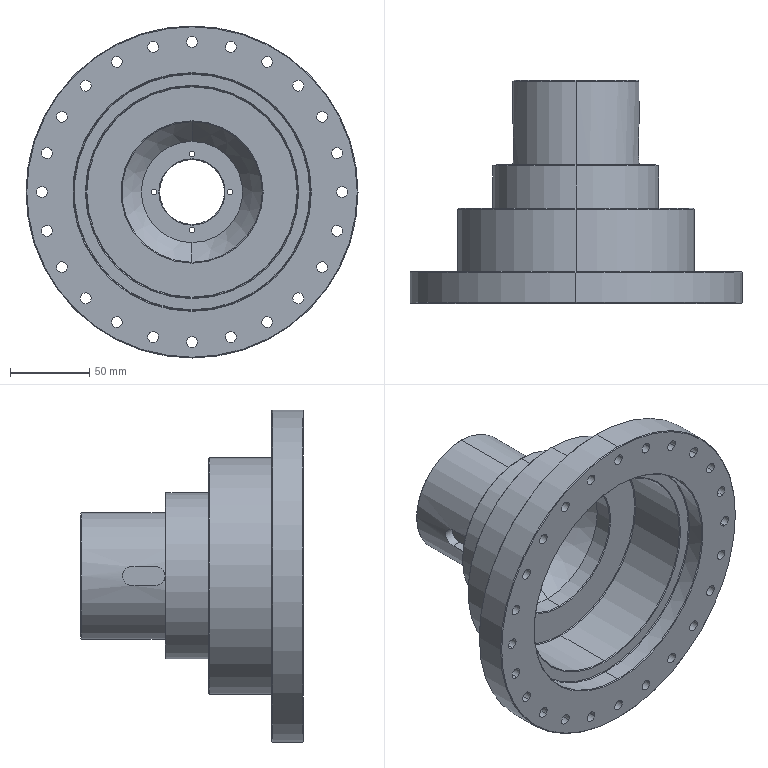CAM job | Mastercam | mm | 3 operations | part box 210 x 141 x 210
1. Drill/Counterbore | 7 - 6 倒角刀
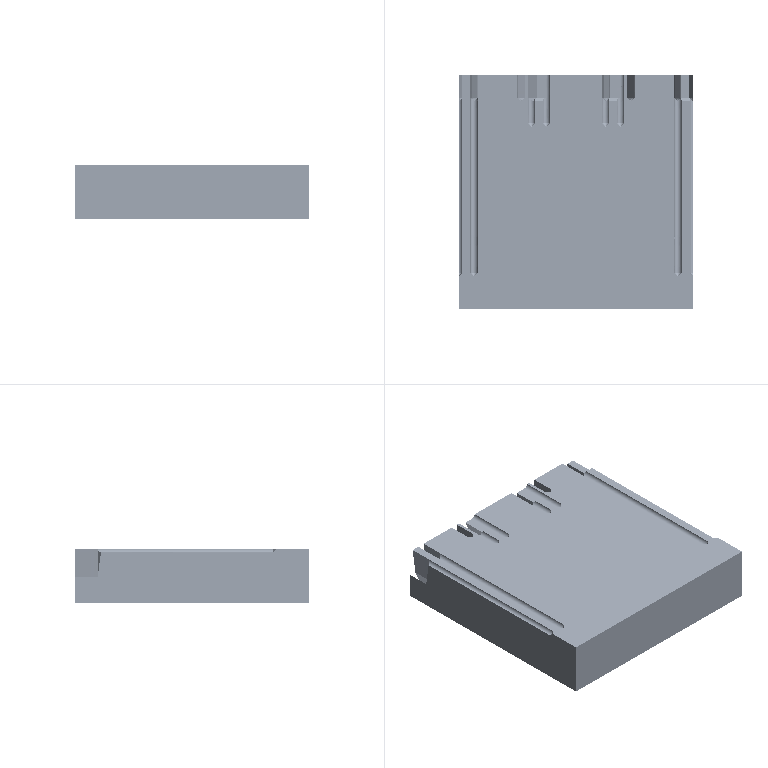2. Contour (Ramp) | 6 - 6 平铣刀
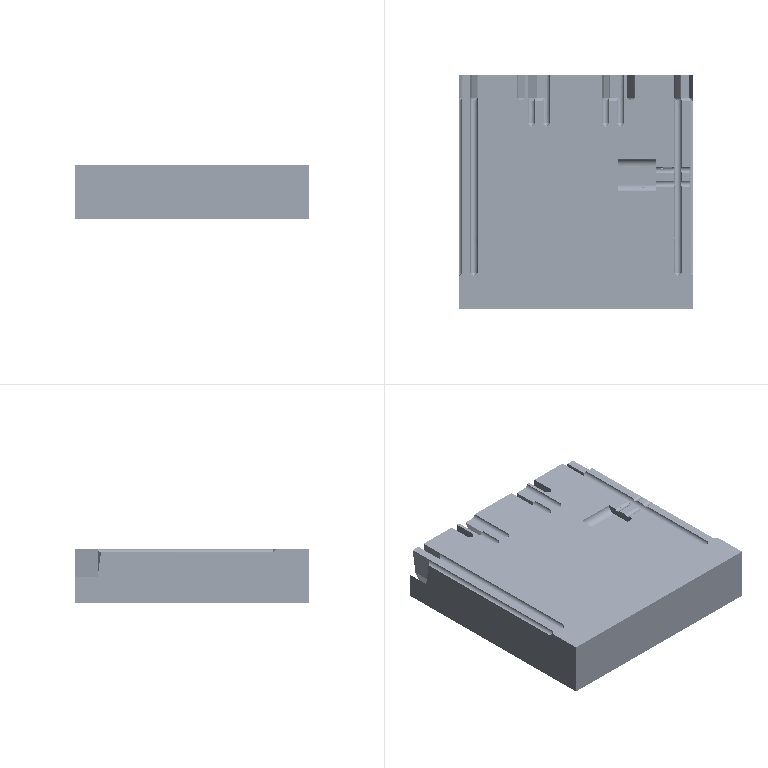3. Contour (2D) | 6 - 6 平铣刀